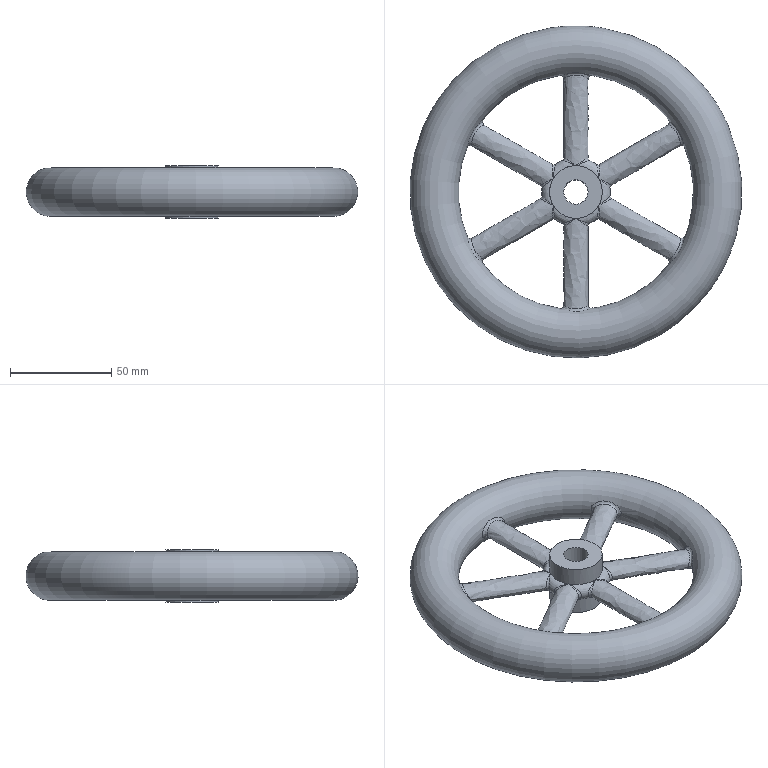Component | NX | 03__HAND_WHEEL__2 | 1 solid | 38 faces | volume 231200 mm3 | spline 18 | torus 9 | other 6 | cylinder 3 | plane 2 | commonest cylinder face diameters 26 x2 12 x1